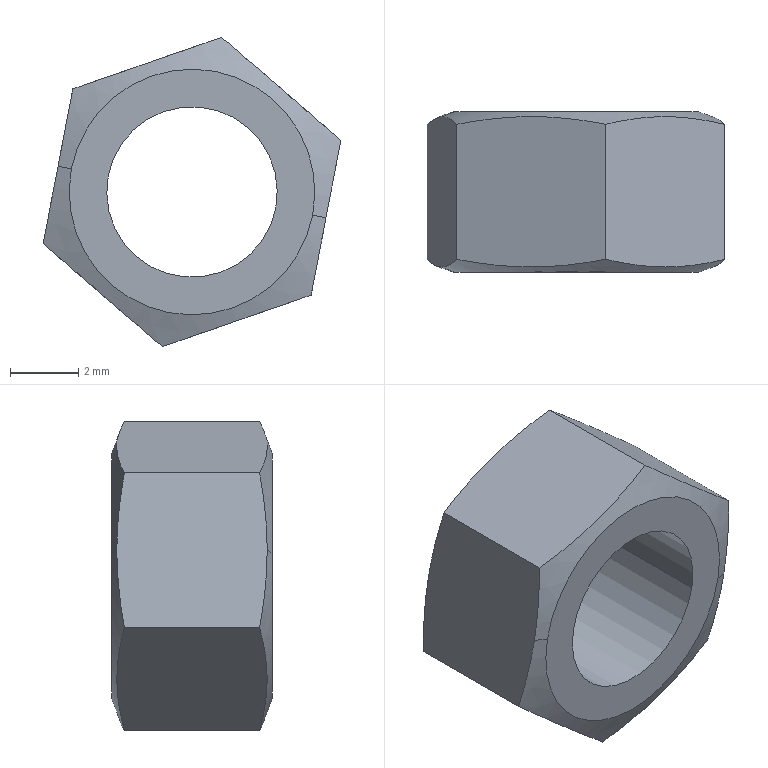Component | SolidWorks | HexNutM5-4 | 1 solid | 14 faces | box 8.73 x 4.7 x 9.07 mm | volume 165 mm3 | plane 8 | cone 4 | cylinder 2 | commonest cylinder face diameters 5 x2
STEP:
#1=COLOUR_RGB('',0.7922,0.8196,0.9333);
#2=FILL_AREA_STYLE_COLOUR('',#1);
#3=FILL_AREA_STYLE('',(#2));
#4=SURFACE_STYLE_FILL_AREA(#3);
#5=SURFACE_SIDE_STYLE('',(#4));
#6=SURFACE_STYLE_USAGE(.BOTH.,#5);
#7=PRESENTATION_STYLE_ASSIGNMENT((#6));
#8=CARTESIAN_POINT('',(-3.847,-0.622,7.213));
#9=VERTEX_POINT('',#8);
#10=CARTESIAN_POINT('',(-3.653,-0.622,7.176));
#11=VERTEX_POINT('',#10);
#12=CARTESIAN_POINT('',(-3.75,-0.622,7.195));
#13=DIRECTION('',(-0.,1.,0.));
#14=DIRECTION('',(0.9821,0.,-0.1885));
#15=AXIS2_PLACEMENT_3D('',#12,#13,#14);
#16=CIRCLE('',#15,0.09843);
#17=EDGE_CURVE('',#9,#11,#16,.T.);
#18=ORIENTED_EDGE('',*,*,#17,.F.);
#19=CARTESIAN_POINT('',(-3.847,-0.437,7.213));
#20=VERTEX_POINT('',#19);
#21=CARTESIAN_POINT('',(-3.847,-0.622,7.213));
#22=DIRECTION('',(-0.,1.,0.));
#23=VECTOR('',#22,39.37);
#24=LINE('',#21,#23);
#25=EDGE_CURVE('',#9,#20,#24,.T.);
#26=ORIENTED_EDGE('',*,*,#25,.T.);
#27=CARTESIAN_POINT('',(-3.653,-0.437,7.176));
#28=VERTEX_POINT('',#27);
#29=CARTESIAN_POINT('',(-3.75,-0.437,7.195));
#30=DIRECTION('',(-0.,1.,0.));
#31=DIRECTION('',(0.9821,0.,-0.1885));
#32=AXIS2_PLACEMENT_3D('',#29,#30,#31);
#33=CIRCLE('',#32,0.09843);
#34=EDGE_CURVE('',#20,#28,#33,.T.);
#35=ORIENTED_EDGE('',*,*,#34,.T.);
#36=CARTESIAN_POINT('',(-3.653,-0.622,7.176));
#37=DIRECTION('',(-0.,1.,0.));
#38=VECTOR('',#37,39.37);
#39=LINE('',#36,#38);
#40=EDGE_CURVE('',#11,#28,#39,.T.);
#41=ORIENTED_EDGE('',*,*,#40,.F.);
#42=EDGE_LOOP('',(#18,#26,#35,#41));
#43=FACE_OUTER_BOUND('',#42,.T.);
#44=CARTESIAN_POINT('',(-3.75,-0.622,7.195));
#45=DIRECTION('',(-0.,1.,0.));
#46=DIRECTION('',(0.9821,0.,-0.1885));
#47=AXIS2_PLACEMENT_3D('',#44,#45,#46);
#48=CYLINDRICAL_SURFACE('',#47,0.09843);
#49=ADVANCED_FACE('',(#43),#48,.F.);
#50=CARTESIAN_POINT('',(-3.889,-0.622,7.222));
#51=VERTEX_POINT('',#50);
#52=CARTESIAN_POINT('',(-3.611,-0.622,7.168));
#53=VERTEX_POINT('',#52);
#54=CARTESIAN_POINT('',(-3.75,-0.622,7.195));
#55=DIRECTION('',(-0.,1.,0.));
#56=DIRECTION('',(0.9821,0.,-0.1885));
#57=AXIS2_PLACEMENT_3D('',#54,#55,#56);
#58=CIRCLE('',#57,0.1417);
#59=EDGE_CURVE('',#51,#53,#58,.T.);
#60=ORIENTED_EDGE('',*,*,#59,.T.);
#61=CARTESIAN_POINT('',(-3.595,-0.6163,7.165));
#62=VERTEX_POINT('',#61);
#63=CARTESIAN_POINT('',(-3.571,-0.6074,7.161));
#64=DIRECTION('',(0.9229,0.342,-0.1771));
#65=VECTOR('',#64,39.37);
#66=LINE('',#63,#65);
#67=EDGE_CURVE('',#53,#62,#66,.T.);
#68=ORIENTED_EDGE('',*,*,#67,.T.);
#69=CARTESIAN_POINT('',(-3.578,-0.6074,7.254));
#70=VERTEX_POINT('',#69);
#71=CARTESIAN_POINT('',(-3.578,-0.6074,7.254));
#72=CARTESIAN_POINT('',(-3.581,-0.6102,7.24));
#73=CARTESIAN_POINT('',(-3.584,-0.6124,7.225));
#74=CARTESIAN_POINT('',(-3.59,-0.6155,7.195));
#75=CARTESIAN_POINT('',(-3.593,-0.6163,7.18));
#76=CARTESIAN_POINT('',(-3.595,-0.6163,7.165));
#77=B_SPLINE_CURVE_WITH_KNOTS('',3,(#71,#72,#73,#74,#75,#76),.UNSPECIFIED.,.F.,.F.,(4,2,4),(0.003914,0.005078,0.006242),.UNSPECIFIED.);
#78=EDGE_CURVE('',#70,#62,#77,.T.);
#79=ORIENTED_EDGE('',*,*,#78,.F.);
#80=CARTESIAN_POINT('',(-3.716,-0.6074,7.373));
#81=VERTEX_POINT('',#80);
#82=CARTESIAN_POINT('',(-3.716,-0.6074,7.373));
#83=CARTESIAN_POINT('',(-3.693,-0.613,7.354));
#84=CARTESIAN_POINT('',(-3.647,-0.6197,7.314));
#85=CARTESIAN_POINT('',(-3.601,-0.613,7.274));
#86=CARTESIAN_POINT('',(-3.578,-0.6074,7.254));
#87=B_SPLINE_CURVE_WITH_KNOTS('',3,(#82,#83,#84,#85,#86),.UNSPECIFIED.,.F.,.F.,(4,1,4),(0.00000023,0.00231,0.004619),.UNSPECIFIED.);
#88=EDGE_CURVE('',#81,#70,#87,.T.);
#89=ORIENTED_EDGE('',*,*,#88,.F.);
#90=CARTESIAN_POINT('',(-3.888,-0.6074,7.314));
#91=VERTEX_POINT('',#90);
#92=CARTESIAN_POINT('',(-3.888,-0.6074,7.314));
#93=CARTESIAN_POINT('',(-3.859,-0.613,7.324));
#94=CARTESIAN_POINT('',(-3.802,-0.6197,7.344));
#95=CARTESIAN_POINT('',(-3.744,-0.613,7.363));
#96=CARTESIAN_POINT('',(-3.716,-0.6074,7.373));
#97=B_SPLINE_CURVE_WITH_KNOTS('',3,(#92,#93,#94,#95,#96),.UNSPECIFIED.,.F.,.F.,(4,1,4),(0.00000023,0.00231,0.004619),.UNSPECIFIED.);
#98=EDGE_CURVE('',#91,#81,#97,.T.);
#99=ORIENTED_EDGE('',*,*,#98,.F.);
#100=CARTESIAN_POINT('',(-3.905,-0.6163,7.225));
#101=VERTEX_POINT('',#100);
#102=CARTESIAN_POINT('',(-3.905,-0.6163,7.225));
#103=CARTESIAN_POINT('',(-3.902,-0.6163,7.239));
#104=CARTESIAN_POINT('',(-3.899,-0.6155,7.254));
#105=CARTESIAN_POINT('',(-3.893,-0.6124,7.284));
#106=CARTESIAN_POINT('',(-3.89,-0.6102,7.299));
#107=CARTESIAN_POINT('',(-3.888,-0.6074,7.314));
#108=B_SPLINE_CURVE_WITH_KNOTS('',3,(#102,#103,#104,#105,#106,#107),.UNSPECIFIED.,.F.,.F.,(4,2,4),(0.01071,0.01187,0.01303),.UNSPECIFIED.);
#109=EDGE_CURVE('',#101,#91,#108,.T.);
#110=ORIENTED_EDGE('',*,*,#109,.F.);
#111=CARTESIAN_POINT('',(-3.929,-0.6074,7.229));
#112=DIRECTION('',(-0.9229,0.342,0.1771));
#113=VECTOR('',#112,39.37);
#114=LINE('',#111,#113);
#115=EDGE_CURVE('',#51,#101,#114,.T.);
#116=ORIENTED_EDGE('',*,*,#115,.F.);
#117=EDGE_LOOP('',(#60,#68,#79,#89,#99,#110,#116));
#118=FACE_OUTER_BOUND('',#117,.T.);
#119=CARTESIAN_POINT('',(-3.75,-0.6074,7.195));
#120=DIRECTION('',(-0.,1.,0.));
#121=DIRECTION('',(-0.9821,0.,0.1885));
#122=AXIS2_PLACEMENT_3D('',#119,#120,#121);
#123=CONICAL_SURFACE('',#122,0.1818,1.222);
#124=ADVANCED_FACE('',(#118),#123,.T.);
#125=CARTESIAN_POINT('',(-3.611,-0.437,7.168));
#126=VERTEX_POINT('',#125);
#127=CARTESIAN_POINT('',(-3.889,-0.437,7.222));
#128=VERTEX_POINT('',#127);
#129=CARTESIAN_POINT('',(-3.75,-0.437,7.195));
#130=DIRECTION('',(-0.,1.,0.));
#131=DIRECTION('',(0.9821,0.,-0.1885));
#132=AXIS2_PLACEMENT_3D('',#129,#130,#131);
#133=CIRCLE('',#132,0.1417);
#134=EDGE_CURVE('',#126,#128,#133,.T.);
#135=ORIENTED_EDGE('',*,*,#134,.F.);
#136=CARTESIAN_POINT('',(-3.595,-0.4427,7.165));
#137=VERTEX_POINT('',#136);
#138=CARTESIAN_POINT('',(-3.571,-0.4516,7.161));
#139=DIRECTION('',(0.9229,-0.342,-0.1771));
#140=VECTOR('',#139,39.37);
#141=LINE('',#138,#140);
#142=EDGE_CURVE('',#126,#137,#141,.T.);
#143=ORIENTED_EDGE('',*,*,#142,.T.);
#144=CARTESIAN_POINT('',(-3.613,-0.4516,7.076));
#145=VERTEX_POINT('',#144);
#146=CARTESIAN_POINT('',(-3.613,-0.4516,7.076));
#147=CARTESIAN_POINT('',(-3.607,-0.4461,7.106));
#148=CARTESIAN_POINT('',(-3.601,-0.4427,7.135));
#149=CARTESIAN_POINT('',(-3.595,-0.4427,7.165));
#150=B_SPLINE_CURVE_WITH_KNOTS('',3,(#146,#147,#148,#149),.UNSPECIFIED.,.F.,.F.,(4,4),(0.008381,0.01071),.UNSPECIFIED.);
#151=EDGE_CURVE('',#145,#137,#150,.T.);
#152=ORIENTED_EDGE('',*,*,#151,.F.);
#153=CARTESIAN_POINT('',(-3.784,-0.4516,7.016));
#154=VERTEX_POINT('',#153);
#155=CARTESIAN_POINT('',(-3.784,-0.4516,7.016));
#156=CARTESIAN_POINT('',(-3.756,-0.4461,7.026));
#157=CARTESIAN_POINT('',(-3.698,-0.4394,7.046));
#158=CARTESIAN_POINT('',(-3.641,-0.4461,7.066));
#159=CARTESIAN_POINT('',(-3.613,-0.4516,7.076));
#160=B_SPLINE_CURVE_WITH_KNOTS('',3,(#155,#156,#157,#158,#159),.UNSPECIFIED.,.F.,.F.,(4,1,4),(0.00000023,0.00231,0.004619),.UNSPECIFIED.);
#161=EDGE_CURVE('',#154,#145,#160,.T.);
#162=ORIENTED_EDGE('',*,*,#161,.F.);
#163=CARTESIAN_POINT('',(-3.922,-0.4516,7.135));
#164=VERTEX_POINT('',#163);
#165=CARTESIAN_POINT('',(-3.922,-0.4516,7.135));
#166=CARTESIAN_POINT('',(-3.899,-0.4461,7.115));
#167=CARTESIAN_POINT('',(-3.853,-0.4394,7.076));
#168=CARTESIAN_POINT('',(-3.807,-0.4461,7.036));
#169=CARTESIAN_POINT('',(-3.784,-0.4516,7.016));
#170=B_SPLINE_CURVE_WITH_KNOTS('',3,(#165,#166,#167,#168,#169),.UNSPECIFIED.,.F.,.F.,(4,1,4),(0.00000023,0.00231,0.004619),.UNSPECIFIED.);
#171=EDGE_CURVE('',#164,#154,#170,.T.);
#172=ORIENTED_EDGE('',*,*,#171,.F.);
#173=CARTESIAN_POINT('',(-3.905,-0.4427,7.225));
#174=VERTEX_POINT('',#173);
#175=CARTESIAN_POINT('',(-3.905,-0.4427,7.225));
#176=CARTESIAN_POINT('',(-3.91,-0.4427,7.195));
#177=CARTESIAN_POINT('',(-3.916,-0.4461,7.165));
#178=CARTESIAN_POINT('',(-3.922,-0.4516,7.135));
#179=B_SPLINE_CURVE_WITH_KNOTS('',3,(#175,#176,#177,#178),.UNSPECIFIED.,.F.,.F.,(4,4),(0.006242,0.008576),.UNSPECIFIED.);
#180=EDGE_CURVE('',#174,#164,#179,.T.);
#181=ORIENTED_EDGE('',*,*,#180,.F.);
#182=CARTESIAN_POINT('',(-3.929,-0.4516,7.229));
#183=DIRECTION('',(-0.9229,-0.342,0.1771));
#184=VECTOR('',#183,39.37);
#185=LINE('',#182,#184);
#186=EDGE_CURVE('',#128,#174,#185,.T.);
#187=ORIENTED_EDGE('',*,*,#186,.F.);
#188=EDGE_LOOP('',(#135,#143,#152,#162,#172,#181,#187));
#189=FACE_OUTER_BOUND('',#188,.T.);
#190=CARTESIAN_POINT('',(-3.75,-0.4516,7.195));
#191=DIRECTION('',(0.,-1.,-0.));
#192=DIRECTION('',(-0.9821,0.,0.1885));
#193=AXIS2_PLACEMENT_3D('',#190,#191,#192);
#194=CONICAL_SURFACE('',#193,0.1818,1.222);
#195=ADVANCED_FACE('',(#189),#194,.T.);
#196=CARTESIAN_POINT('',(-3.613,-0.6074,7.076));
#197=VERTEX_POINT('',#196);
#198=CARTESIAN_POINT('',(-3.613,-0.437,7.076));
#199=DIRECTION('',(0.,-1.,-0.));
#200=VECTOR('',#199,39.37);
#201=LINE('',#198,#200);
#202=EDGE_CURVE('',#145,#197,#201,.T.);
#203=ORIENTED_EDGE('',*,*,#202,.T.);
#204=CARTESIAN_POINT('',(-3.784,-0.6074,7.016));
#205=VERTEX_POINT('',#204);
#206=CARTESIAN_POINT('',(-3.613,-0.6074,7.076));
#207=CARTESIAN_POINT('',(-3.641,-0.613,7.066));
#208=CARTESIAN_POINT('',(-3.698,-0.6197,7.046));
#209=CARTESIAN_POINT('',(-3.756,-0.613,7.026));
#210=CARTESIAN_POINT('',(-3.784,-0.6074,7.016));
#211=B_SPLINE_CURVE_WITH_KNOTS('',3,(#206,#207,#208,#209,#210),.UNSPECIFIED.,.F.,.F.,(4,1,4),(0.00000023,0.00231,0.004619),.UNSPECIFIED.);
#212=EDGE_CURVE('',#197,#205,#211,.T.);
#213=ORIENTED_EDGE('',*,*,#212,.T.);
#214=CARTESIAN_POINT('',(-3.784,-0.437,7.016));
#215=DIRECTION('',(0.,-1.,-0.));
#216=VECTOR('',#215,39.37);
#217=LINE('',#214,#216);
#218=EDGE_CURVE('',#154,#205,#217,.T.);
#219=ORIENTED_EDGE('',*,*,#218,.F.);
#220=ORIENTED_EDGE('',*,*,#161,.T.);
#221=EDGE_LOOP('',(#203,#213,#219,#220));
#222=FACE_OUTER_BOUND('',#221,.T.);
#223=CARTESIAN_POINT('',(-3.613,-0.437,7.076));
#224=DIRECTION('',(-0.3278,-0.,0.9447));
#225=DIRECTION('',(0.9447,0.,0.3278));
#226=AXIS2_PLACEMENT_3D('',#223,#224,#225);
#227=PLANE('',#226);
#228=ADVANCED_FACE('',(#222),#227,.F.);
#229=ORIENTED_EDGE('',*,*,#218,.T.);
#230=CARTESIAN_POINT('',(-3.922,-0.6074,7.135));
#231=VERTEX_POINT('',#230);
#232=CARTESIAN_POINT('',(-3.784,-0.6074,7.016));
#233=CARTESIAN_POINT('',(-3.807,-0.613,7.036));
#234=CARTESIAN_POINT('',(-3.853,-0.6197,7.076));
#235=CARTESIAN_POINT('',(-3.899,-0.613,7.115));
#236=CARTESIAN_POINT('',(-3.922,-0.6074,7.135));
#237=B_SPLINE_CURVE_WITH_KNOTS('',3,(#232,#233,#234,#235,#236),.UNSPECIFIED.,.F.,.F.,(4,1,4),(0.00000023,0.00231,0.004619),.UNSPECIFIED.);
#238=EDGE_CURVE('',#205,#231,#237,.T.);
#239=ORIENTED_EDGE('',*,*,#238,.T.);
#240=CARTESIAN_POINT('',(-3.922,-0.437,7.135));
#241=DIRECTION('',(0.,-1.,-0.));
#242=VECTOR('',#241,39.37);
#243=LINE('',#240,#242);
#244=EDGE_CURVE('',#164,#231,#243,.T.);
#245=ORIENTED_EDGE('',*,*,#244,.F.);
#246=ORIENTED_EDGE('',*,*,#171,.T.);
#247=EDGE_LOOP('',(#229,#239,#245,#246));
#248=FACE_OUTER_BOUND('',#247,.T.);
#249=CARTESIAN_POINT('',(-3.784,-0.437,7.016));
#250=DIRECTION('',(0.6542,0.,0.7563));
#251=DIRECTION('',(0.7563,0.,-0.6542));
#252=AXIS2_PLACEMENT_3D('',#249,#250,#251);
#253=PLANE('',#252);
#254=ADVANCED_FACE('',(#248),#253,.F.);
#255=ORIENTED_EDGE('',*,*,#244,.T.);
#256=CARTESIAN_POINT('',(-3.922,-0.6074,7.135));
#257=CARTESIAN_POINT('',(-3.916,-0.6129,7.165));
#258=CARTESIAN_POINT('',(-3.91,-0.6163,7.195));
#259=CARTESIAN_POINT('',(-3.905,-0.6163,7.225));
#260=B_SPLINE_CURVE_WITH_KNOTS('',3,(#256,#257,#258,#259),.UNSPECIFIED.,.F.,.F.,(4,4),(0.008381,0.01071),.UNSPECIFIED.);
#261=EDGE_CURVE('',#231,#101,#260,.T.);
#262=ORIENTED_EDGE('',*,*,#261,.T.);
#263=ORIENTED_EDGE('',*,*,#109,.T.);
#264=CARTESIAN_POINT('',(-3.888,-0.4516,7.314));
#265=VERTEX_POINT('',#264);
#266=CARTESIAN_POINT('',(-3.888,-0.437,7.314));
#267=DIRECTION('',(0.,-1.,-0.));
#268=VECTOR('',#267,39.37);
#269=LINE('',#266,#268);
#270=EDGE_CURVE('',#265,#91,#269,.T.);
#271=ORIENTED_EDGE('',*,*,#270,.F.);
#272=CARTESIAN_POINT('',(-3.888,-0.4516,7.314));
#273=CARTESIAN_POINT('',(-3.89,-0.4489,7.299));
#274=CARTESIAN_POINT('',(-3.893,-0.4466,7.284));
#275=CARTESIAN_POINT('',(-3.899,-0.4435,7.254));
#276=CARTESIAN_POINT('',(-3.902,-0.4427,7.239));
#277=CARTESIAN_POINT('',(-3.905,-0.4427,7.225));
#278=B_SPLINE_CURVE_WITH_KNOTS('',3,(#272,#273,#274,#275,#276,#277),.UNSPECIFIED.,.F.,.F.,(4,2,4),(0.003914,0.005078,0.006242),.UNSPECIFIED.);
#279=EDGE_CURVE('',#265,#174,#278,.T.);
#280=ORIENTED_EDGE('',*,*,#279,.T.);
#281=ORIENTED_EDGE('',*,*,#180,.T.);
#282=EDGE_LOOP('',(#255,#262,#263,#271,#280,#281));
#283=FACE_OUTER_BOUND('',#282,.T.);
#284=CARTESIAN_POINT('',(-3.922,-0.437,7.135));
#285=DIRECTION('',(0.9821,0.,-0.1885));
#286=DIRECTION('',(0.,-1.,-0.));
#287=AXIS2_PLACEMENT_3D('',#284,#285,#286);
#288=PLANE('',#287);
#289=ADVANCED_FACE('',(#283),#288,.F.);
#290=ORIENTED_EDGE('',*,*,#270,.T.);
#291=ORIENTED_EDGE('',*,*,#98,.T.);
#292=CARTESIAN_POINT('',(-3.716,-0.4516,7.373));
#293=VERTEX_POINT('',#292);
#294=CARTESIAN_POINT('',(-3.716,-0.437,7.373));
#295=DIRECTION('',(0.,-1.,-0.));
#296=VECTOR('',#295,39.37);
#297=LINE('',#294,#296);
#298=EDGE_CURVE('',#293,#81,#297,.T.);
#299=ORIENTED_EDGE('',*,*,#298,.F.);
#300=CARTESIAN_POINT('',(-3.716,-0.4516,7.373));
#301=CARTESIAN_POINT('',(-3.744,-0.4461,7.363));
#302=CARTESIAN_POINT('',(-3.802,-0.4394,7.344));
#303=CARTESIAN_POINT('',(-3.859,-0.4461,7.324));
#304=CARTESIAN_POINT('',(-3.888,-0.4516,7.314));
#305=B_SPLINE_CURVE_WITH_KNOTS('',3,(#300,#301,#302,#303,#304),.UNSPECIFIED.,.F.,.F.,(4,1,4),(0.00000023,0.00231,0.004619),.UNSPECIFIED.);
#306=EDGE_CURVE('',#293,#265,#305,.T.);
#307=ORIENTED_EDGE('',*,*,#306,.T.);
#308=EDGE_LOOP('',(#290,#291,#299,#307));
#309=FACE_OUTER_BOUND('',#308,.T.);
#310=CARTESIAN_POINT('',(-3.888,-0.437,7.314));
#311=DIRECTION('',(0.3278,0.,-0.9447));
#312=DIRECTION('',(-0.9447,-0.,-0.3278));
#313=AXIS2_PLACEMENT_3D('',#310,#311,#312);
#314=PLANE('',#313);
#315=ADVANCED_FACE('',(#309),#314,.F.);
#316=ORIENTED_EDGE('',*,*,#298,.T.);
#317=ORIENTED_EDGE('',*,*,#88,.T.);
#318=CARTESIAN_POINT('',(-3.578,-0.4516,7.254));
#319=VERTEX_POINT('',#318);
#320=CARTESIAN_POINT('',(-3.578,-0.437,7.254));
#321=DIRECTION('',(0.,-1.,-0.));
#322=VECTOR('',#321,39.37);
#323=LINE('',#320,#322);
#324=EDGE_CURVE('',#319,#70,#323,.T.);
#325=ORIENTED_EDGE('',*,*,#324,.F.);
#326=CARTESIAN_POINT('',(-3.578,-0.4516,7.254));
#327=CARTESIAN_POINT('',(-3.601,-0.4461,7.274));
#328=CARTESIAN_POINT('',(-3.647,-0.4394,7.314));
#329=CARTESIAN_POINT('',(-3.693,-0.4461,7.354));
#330=CARTESIAN_POINT('',(-3.716,-0.4516,7.373));
#331=B_SPLINE_CURVE_WITH_KNOTS('',3,(#326,#327,#328,#329,#330),.UNSPECIFIED.,.F.,.F.,(4,1,4),(0.00000023,0.00231,0.004619),.UNSPECIFIED.);
#332=EDGE_CURVE('',#319,#293,#331,.T.);
#333=ORIENTED_EDGE('',*,*,#332,.T.);
#334=EDGE_LOOP('',(#316,#317,#325,#333));
#335=FACE_OUTER_BOUND('',#334,.T.);
#336=CARTESIAN_POINT('',(-3.716,-0.437,7.373));
#337=DIRECTION('',(-0.6542,-0.,-0.7563));
#338=DIRECTION('',(-0.7563,-0.,0.6542));
#339=AXIS2_PLACEMENT_3D('',#336,#337,#338);
#340=PLANE('',#339);
#341=ADVANCED_FACE('',(#335),#340,.F.);
#342=ORIENTED_EDGE('',*,*,#324,.T.);
#343=ORIENTED_EDGE('',*,*,#78,.T.);
#344=CARTESIAN_POINT('',(-3.595,-0.6163,7.165));
#345=CARTESIAN_POINT('',(-3.601,-0.6163,7.135));
#346=CARTESIAN_POINT('',(-3.607,-0.6129,7.106));
#347=CARTESIAN_POINT('',(-3.613,-0.6074,7.076));
#348=B_SPLINE_CURVE_WITH_KNOTS('',3,(#344,#345,#346,#347),.UNSPECIFIED.,.F.,.F.,(4,4),(0.006242,0.008576),.UNSPECIFIED.);
#349=EDGE_CURVE('',#62,#197,#348,.T.);
#350=ORIENTED_EDGE('',*,*,#349,.T.);
#351=ORIENTED_EDGE('',*,*,#202,.F.);
#352=ORIENTED_EDGE('',*,*,#151,.T.);
#353=CARTESIAN_POINT('',(-3.595,-0.4427,7.165));
#354=CARTESIAN_POINT('',(-3.593,-0.4427,7.18));
#355=CARTESIAN_POINT('',(-3.59,-0.4435,7.195));
#356=CARTESIAN_POINT('',(-3.584,-0.4466,7.225));
#357=CARTESIAN_POINT('',(-3.581,-0.4489,7.24));
#358=CARTESIAN_POINT('',(-3.578,-0.4516,7.254));
#359=B_SPLINE_CURVE_WITH_KNOTS('',3,(#353,#354,#355,#356,#357,#358),.UNSPECIFIED.,.F.,.F.,(4,2,4),(0.01071,0.01187,0.01303),.UNSPECIFIED.);
#360=EDGE_CURVE('',#137,#319,#359,.T.);
#361=ORIENTED_EDGE('',*,*,#360,.T.);
#362=EDGE_LOOP('',(#342,#343,#350,#351,#352,#361));
#363=FACE_OUTER_BOUND('',#362,.T.);
#364=CARTESIAN_POINT('',(-3.578,-0.437,7.254));
#365=DIRECTION('',(-0.9821,-0.,0.1885));
#366=DIRECTION('',(-0.,1.,0.));
#367=AXIS2_PLACEMENT_3D('',#364,#365,#366);
#368=PLANE('',#367);
#369=ADVANCED_FACE('',(#363),#368,.F.);
#370=ORIENTED_EDGE('',*,*,#142,.F.);
#371=CARTESIAN_POINT('',(-3.75,-0.437,7.195));
#372=DIRECTION('',(-0.,1.,0.));
#373=DIRECTION('',(0.9821,0.,-0.1885));
#374=AXIS2_PLACEMENT_3D('',#371,#372,#373);
#375=CIRCLE('',#374,0.1417);
#376=EDGE_CURVE('',#128,#126,#375,.T.);
#377=ORIENTED_EDGE('',*,*,#376,.F.);
#378=ORIENTED_EDGE('',*,*,#186,.T.);
#379=ORIENTED_EDGE('',*,*,#279,.F.);
#380=ORIENTED_EDGE('',*,*,#306,.F.);
#381=ORIENTED_EDGE('',*,*,#332,.F.);
#382=ORIENTED_EDGE('',*,*,#360,.F.);
#383=EDGE_LOOP('',(#370,#377,#378,#379,#380,#381,#382));
#384=FACE_OUTER_BOUND('',#383,.T.);
#385=CARTESIAN_POINT('',(-3.75,-0.4516,7.195));
#386=DIRECTION('',(0.,-1.,-0.));
#387=DIRECTION('',(-0.9821,0.,0.1885));
#388=AXIS2_PLACEMENT_3D('',#385,#386,#387);
#389=CONICAL_SURFACE('',#388,0.1818,1.222);
#390=ADVANCED_FACE('',(#384),#389,.T.);
#391=CARTESIAN_POINT('',(-3.75,-0.437,7.195));
#392=DIRECTION('',(-0.,1.,0.));
#393=DIRECTION('',(0.9821,0.,-0.1885));
#394=AXIS2_PLACEMENT_3D('',#391,#392,#393);
#395=CIRCLE('',#394,0.09843);
#396=EDGE_CURVE('',#28,#20,#395,.T.);
#397=ORIENTED_EDGE('',*,*,#396,.F.);
#398=ORIENTED_EDGE('',*,*,#34,.F.);
#399=EDGE_LOOP('',(#397,#398));
#400=FACE_BOUND('',#399,.T.);
#401=ORIENTED_EDGE('',*,*,#376,.T.);
#402=ORIENTED_EDGE('',*,*,#134,.T.);
#403=EDGE_LOOP('',(#401,#402));
#404=FACE_OUTER_BOUND('',#403,.T.);
#405=CARTESIAN_POINT('',(-3.75,-0.437,7.195));
#406=DIRECTION('',(-0.,1.,0.));
#407=DIRECTION('',(0.9821,0.,-0.1885));
#408=AXIS2_PLACEMENT_3D('',#405,#406,#407);
#409=PLANE('',#408);
#410=ADVANCED_FACE('',(#400,#404),#409,.T.);
#411=ORIENTED_EDGE('',*,*,#67,.F.);
#412=CARTESIAN_POINT('',(-3.75,-0.622,7.195));
#413=DIRECTION('',(-0.,1.,0.));
#414=DIRECTION('',(0.9821,0.,-0.1885));
#415=AXIS2_PLACEMENT_3D('',#412,#413,#414);
#416=CIRCLE('',#415,0.1417);
#417=EDGE_CURVE('',#53,#51,#416,.T.);
#418=ORIENTED_EDGE('',*,*,#417,.T.);
#419=ORIENTED_EDGE('',*,*,#115,.T.);
#420=ORIENTED_EDGE('',*,*,#261,.F.);
#421=ORIENTED_EDGE('',*,*,#238,.F.);
#422=ORIENTED_EDGE('',*,*,#212,.F.);
#423=ORIENTED_EDGE('',*,*,#349,.F.);
#424=EDGE_LOOP('',(#411,#418,#419,#420,#421,#422,#423));
#425=FACE_OUTER_BOUND('',#424,.T.);
#426=CARTESIAN_POINT('',(-3.75,-0.6074,7.195));
#427=DIRECTION('',(-0.,1.,0.));
#428=DIRECTION('',(-0.9821,0.,0.1885));
#429=AXIS2_PLACEMENT_3D('',#426,#427,#428);
#430=CONICAL_SURFACE('',#429,0.1818,1.222);
#431=ADVANCED_FACE('',(#425),#430,.T.);
#432=CARTESIAN_POINT('',(-3.75,-0.622,7.195));
#433=DIRECTION('',(-0.,1.,0.));
#434=DIRECTION('',(0.9821,0.,-0.1885));
#435=AXIS2_PLACEMENT_3D('',#432,#433,#434);
#436=CIRCLE('',#435,0.09843);
#437=EDGE_CURVE('',#11,#9,#436,.T.);
#438=ORIENTED_EDGE('',*,*,#437,.T.);
#439=ORIENTED_EDGE('',*,*,#17,.T.);
#440=EDGE_LOOP('',(#438,#439));
#441=FACE_BOUND('',#440,.T.);
#442=ORIENTED_EDGE('',*,*,#59,.F.);
#443=ORIENTED_EDGE('',*,*,#417,.F.);
#444=EDGE_LOOP('',(#442,#443));
#445=FACE_OUTER_BOUND('',#444,.T.);
#446=CARTESIAN_POINT('',(-3.75,-0.622,7.195));
#447=DIRECTION('',(-0.,1.,0.));
#448=DIRECTION('',(0.9821,0.,-0.1885));
#449=AXIS2_PLACEMENT_3D('',#446,#447,#448);
#450=PLANE('',#449);
#451=ADVANCED_FACE('',(#441,#445),#450,.F.);
#452=ORIENTED_EDGE('',*,*,#25,.F.);
#453=ORIENTED_EDGE('',*,*,#437,.F.);
#454=ORIENTED_EDGE('',*,*,#40,.T.);
#455=ORIENTED_EDGE('',*,*,#396,.T.);
#456=EDGE_LOOP('',(#452,#453,#454,#455));
#457=FACE_OUTER_BOUND('',#456,.T.);
#458=CARTESIAN_POINT('',(-3.75,-0.622,7.195));
#459=DIRECTION('',(-0.,1.,0.));
#460=DIRECTION('',(0.9821,0.,-0.1885));
#461=AXIS2_PLACEMENT_3D('',#458,#459,#460);
#462=CYLINDRICAL_SURFACE('',#461,0.09843);
#463=ADVANCED_FACE('',(#457),#462,.F.);
#464=CLOSED_SHELL('',(#49,#124,#195,#228,#254,#289,#315,#341,#369,#390,#410,#431,#451,#463));
#465=MANIFOLD_SOLID_BREP('',#464);
#466=STYLED_ITEM('',(#7),#465);
#467=(LENGTH_UNIT()NAMED_UNIT(*)SI_UNIT($,.METRE.));
#468=LENGTH_MEASURE_WITH_UNIT(LENGTH_MEASURE(0.0254),#467);
#469=DIMENSIONAL_EXPONENTS(1.,0.,0.,0.,0.,0.,0.);
#470=(CONVERSION_BASED_UNIT('',#468)LENGTH_UNIT()NAMED_UNIT(#469));
#471=UNCERTAINTY_MEASURE_WITH_UNIT(LENGTH_MEASURE(0.00001),#470,'','');
#472=(NAMED_UNIT(*)PLANE_ANGLE_UNIT()SI_UNIT($,.RADIAN.));
#473=(NAMED_UNIT(*)SI_UNIT($,.STERADIAN.)SOLID_ANGLE_UNIT());
#474=(GEOMETRIC_REPRESENTATION_CONTEXT(3)GLOBAL_UNCERTAINTY_ASSIGNED_CONTEXT((#471))GLOBAL_UNIT_ASSIGNED_CONTEXT((#470,#472,#473))REPRESENTATION_CONTEXT('',''));
#475=MECHANICAL_DESIGN_GEOMETRIC_PRESENTATION_REPRESENTATION('',(#466),#474);
#476=PRESENTATION_LAYER_ASSIGNMENT('','',(#466));
#477=CARTESIAN_POINT('',(0.,0.,0.));
#478=DIRECTION('',(0.,0.,1.));
#479=DIRECTION('',(1.,0.,0.));
#480=AXIS2_PLACEMENT_3D('',#477,#478,#479);
#481=(LENGTH_UNIT()NAMED_UNIT(*)SI_UNIT($,.METRE.));
#482=LENGTH_MEASURE_WITH_UNIT(LENGTH_MEASURE(0.0254),#481);
#483=DIMENSIONAL_EXPONENTS(1.,0.,0.,0.,0.,0.,0.);
#484=(CONVERSION_BASED_UNIT('',#482)LENGTH_UNIT()NAMED_UNIT(#483));
#485=UNCERTAINTY_MEASURE_WITH_UNIT(LENGTH_MEASURE(0.00001),#484,'','');
#486=(NAMED_UNIT(*)PLANE_ANGLE_UNIT()SI_UNIT($,.RADIAN.));
#487=(NAMED_UNIT(*)SI_UNIT($,.STERADIAN.)SOLID_ANGLE_UNIT());
#488=(GEOMETRIC_REPRESENTATION_CONTEXT(3)GLOBAL_UNCERTAINTY_ASSIGNED_CONTEXT((#485))GLOBAL_UNIT_ASSIGNED_CONTEXT((#484,#486,#487))REPRESENTATION_CONTEXT('',''));
#489=ADVANCED_BREP_SHAPE_REPRESENTATION('',(#465,#480),#488);